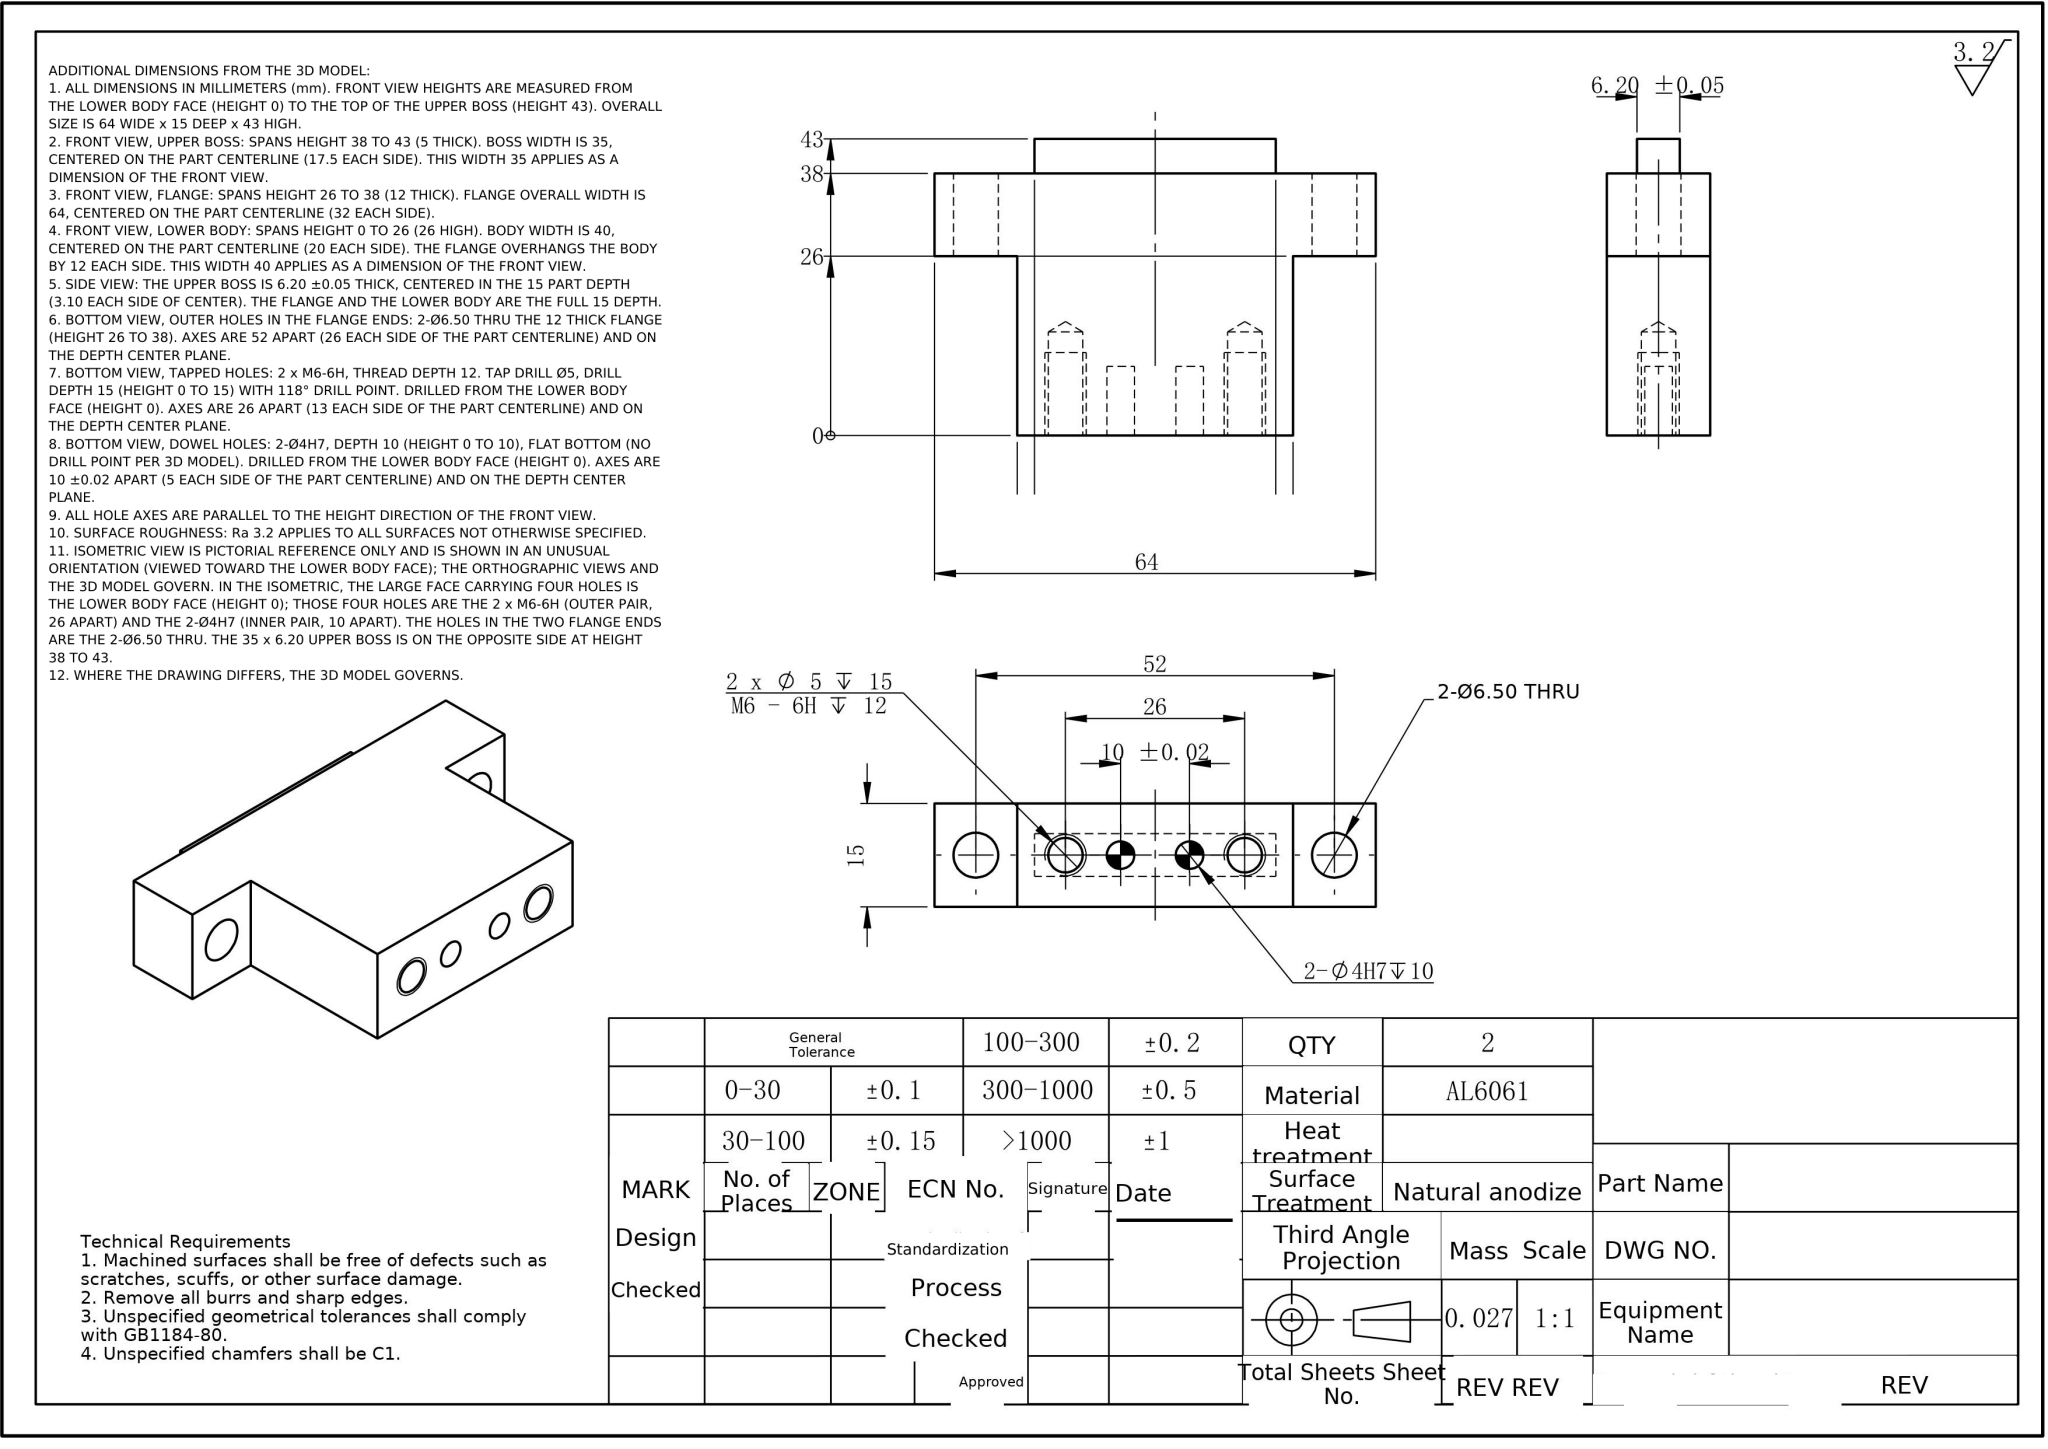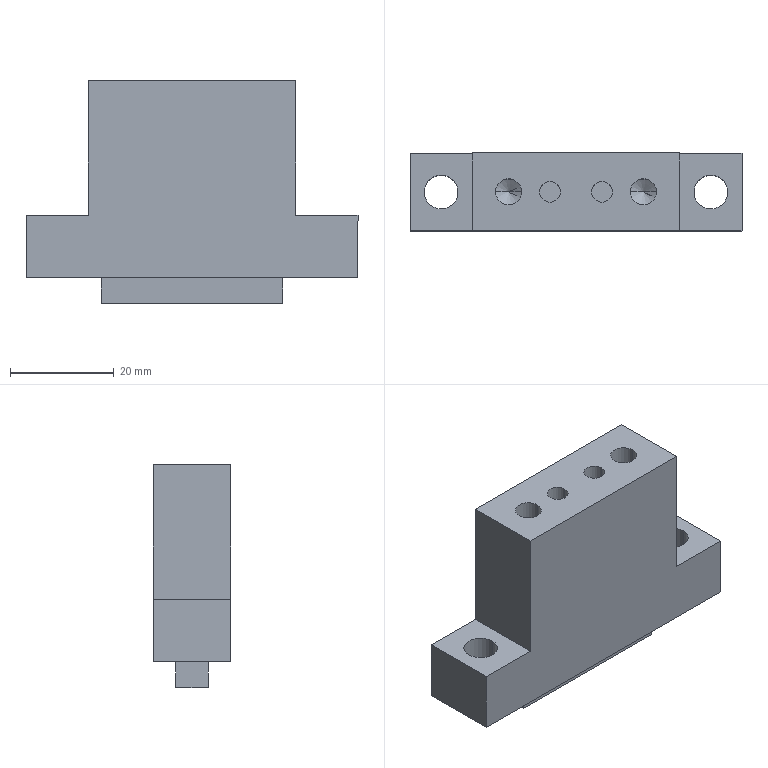Part | NX | mm | 1 solid | 33 faces | box 64 x 15 x 43 mm | volume 26549 mm3 | plane 17 | cylinder 12 | cone 4 | commonest cylinder face diameters 4 x4 5 x4 6.5 x4
STEP:
#1=CARTESIAN_POINT('',(-7.,-0.,-52.75));
#2=VERTEX_POINT('',#1);
#3=CARTESIAN_POINT('',(-3.,-0.,-52.75));
#4=VERTEX_POINT('',#3);
#5=CARTESIAN_POINT('',(-5.,-0.,-52.75));
#6=DIRECTION('',(0.,0.,1.));
#7=DIRECTION('',(-1.,0.,0.));
#8=AXIS2_PLACEMENT_3D('',#5,#6,#7);
#9=CIRCLE('',#8,2.);
#10=EDGE_CURVE('',#2,#4,#9,.T.);
#11=ORIENTED_EDGE('',*,*,#10,.F.);
#12=CARTESIAN_POINT('',(-7.,-0.,-42.75));
#13=VERTEX_POINT('',#12);
#14=CARTESIAN_POINT('',(-7.,-0.,-52.75));
#15=DIRECTION('',(0.,0.,1.));
#16=VECTOR('',#15,1000.);
#17=LINE('',#14,#16);
#18=EDGE_CURVE('',#2,#13,#17,.T.);
#19=ORIENTED_EDGE('',*,*,#18,.T.);
#20=CARTESIAN_POINT('',(-3.,-0.,-42.75));
#21=VERTEX_POINT('',#20);
#22=CARTESIAN_POINT('',(-5.,-0.,-42.75));
#23=DIRECTION('',(0.,0.,1.));
#24=DIRECTION('',(-1.,0.,0.));
#25=AXIS2_PLACEMENT_3D('',#22,#23,#24);
#26=CIRCLE('',#25,2.);
#27=EDGE_CURVE('',#13,#21,#26,.T.);
#28=ORIENTED_EDGE('',*,*,#27,.T.);
#29=CARTESIAN_POINT('',(-3.,-0.,-52.75));
#30=DIRECTION('',(0.,0.,1.));
#31=VECTOR('',#30,1000.);
#32=LINE('',#29,#31);
#33=EDGE_CURVE('',#4,#21,#32,.T.);
#34=ORIENTED_EDGE('',*,*,#33,.F.);
#35=EDGE_LOOP('',(#11,#19,#28,#34));
#36=FACE_OUTER_BOUND('',#35,.T.);
#37=CARTESIAN_POINT('',(-5.,-0.,-52.75));
#38=DIRECTION('',(0.,0.,1.));
#39=DIRECTION('',(1.,0.,0.));
#40=AXIS2_PLACEMENT_3D('',#37,#38,#39);
#41=CYLINDRICAL_SURFACE('',#40,2.);
#42=ADVANCED_FACE('',(#36),#41,.F.);
#43=CARTESIAN_POINT('',(3.,0.,-52.75));
#44=VERTEX_POINT('',#43);
#45=CARTESIAN_POINT('',(7.,0.,-52.75));
#46=VERTEX_POINT('',#45);
#47=CARTESIAN_POINT('',(5.,0.,-52.75));
#48=DIRECTION('',(0.,0.,1.));
#49=DIRECTION('',(1.,0.,0.));
#50=AXIS2_PLACEMENT_3D('',#47,#48,#49);
#51=CIRCLE('',#50,2.);
#52=EDGE_CURVE('',#44,#46,#51,.T.);
#53=ORIENTED_EDGE('',*,*,#52,.F.);
#54=CARTESIAN_POINT('',(3.,0.,-42.75));
#55=VERTEX_POINT('',#54);
#56=CARTESIAN_POINT('',(3.,0.,-52.75));
#57=DIRECTION('',(0.,0.,1.));
#58=VECTOR('',#57,1000.);
#59=LINE('',#56,#58);
#60=EDGE_CURVE('',#44,#55,#59,.T.);
#61=ORIENTED_EDGE('',*,*,#60,.T.);
#62=CARTESIAN_POINT('',(7.,0.,-42.75));
#63=VERTEX_POINT('',#62);
#64=CARTESIAN_POINT('',(5.,0.,-42.75));
#65=DIRECTION('',(0.,0.,1.));
#66=DIRECTION('',(1.,0.,0.));
#67=AXIS2_PLACEMENT_3D('',#64,#65,#66);
#68=CIRCLE('',#67,2.);
#69=EDGE_CURVE('',#55,#63,#68,.T.);
#70=ORIENTED_EDGE('',*,*,#69,.T.);
#71=CARTESIAN_POINT('',(7.,0.,-52.75));
#72=DIRECTION('',(0.,0.,1.));
#73=VECTOR('',#72,1000.);
#74=LINE('',#71,#73);
#75=EDGE_CURVE('',#46,#63,#74,.T.);
#76=ORIENTED_EDGE('',*,*,#75,.F.);
#77=EDGE_LOOP('',(#53,#61,#70,#76));
#78=FACE_OUTER_BOUND('',#77,.T.);
#79=CARTESIAN_POINT('',(5.,0.,-52.75));
#80=DIRECTION('',(0.,0.,1.));
#81=DIRECTION('',(1.,0.,0.));
#82=AXIS2_PLACEMENT_3D('',#79,#80,#81);
#83=CYLINDRICAL_SURFACE('',#82,2.);
#84=ADVANCED_FACE('',(#78),#83,.F.);
#85=CARTESIAN_POINT('',(10.5,0.,-57.75));
#86=VERTEX_POINT('',#85);
#87=CARTESIAN_POINT('',(15.5,0.,-57.75));
#88=VERTEX_POINT('',#87);
#89=CARTESIAN_POINT('',(13.,0.,-57.75));
#90=DIRECTION('',(0.,0.,1.));
#91=DIRECTION('',(1.,0.,0.));
#92=AXIS2_PLACEMENT_3D('',#89,#90,#91);
#93=CIRCLE('',#92,2.5);
#94=EDGE_CURVE('',#86,#88,#93,.T.);
#95=ORIENTED_EDGE('',*,*,#94,.F.);
#96=CARTESIAN_POINT('',(10.5,0.,-42.75));
#97=VERTEX_POINT('',#96);
#98=CARTESIAN_POINT('',(10.5,0.,-42.75));
#99=DIRECTION('',(0.,0.,1.));
#100=VECTOR('',#99,1000.);
#101=LINE('',#98,#100);
#102=EDGE_CURVE('',#86,#97,#101,.T.);
#103=ORIENTED_EDGE('',*,*,#102,.T.);
#104=CARTESIAN_POINT('',(15.5,0.,-42.75));
#105=VERTEX_POINT('',#104);
#106=CARTESIAN_POINT('',(13.,0.,-42.75));
#107=DIRECTION('',(0.,0.,1.));
#108=DIRECTION('',(1.,0.,0.));
#109=AXIS2_PLACEMENT_3D('',#106,#107,#108);
#110=CIRCLE('',#109,2.5);
#111=EDGE_CURVE('',#97,#105,#110,.T.);
#112=ORIENTED_EDGE('',*,*,#111,.T.);
#113=CARTESIAN_POINT('',(15.5,0.,-42.75));
#114=DIRECTION('',(0.,0.,1.));
#115=VECTOR('',#114,1000.);
#116=LINE('',#113,#115);
#117=EDGE_CURVE('',#88,#105,#116,.T.);
#118=ORIENTED_EDGE('',*,*,#117,.F.);
#119=EDGE_LOOP('',(#95,#103,#112,#118));
#120=FACE_OUTER_BOUND('',#119,.T.);
#121=CARTESIAN_POINT('',(13.,0.,-42.75));
#122=DIRECTION('',(0.,0.,1.));
#123=DIRECTION('',(1.,0.,0.));
#124=AXIS2_PLACEMENT_3D('',#121,#122,#123);
#125=CYLINDRICAL_SURFACE('',#124,2.5);
#126=ADVANCED_FACE('',(#120),#125,.F.);
#127=CARTESIAN_POINT('',(13.,0.,-59.252));
#128=VERTEX_POINT('',#127);
#129=CARTESIAN_POINT('',(15.5,0.,-57.75));
#130=DIRECTION('',(0.8572,0.,0.515));
#131=VECTOR('',#130,1000.);
#132=LINE('',#129,#131);
#133=EDGE_CURVE('',#128,#88,#132,.T.);
#134=ORIENTED_EDGE('',*,*,#133,.F.);
#135=CARTESIAN_POINT('',(10.5,0.,-57.75));
#136=DIRECTION('',(-0.8572,0.,0.515));
#137=VECTOR('',#136,1000.);
#138=LINE('',#135,#137);
#139=EDGE_CURVE('',#128,#86,#138,.T.);
#140=ORIENTED_EDGE('',*,*,#139,.T.);
#141=ORIENTED_EDGE('',*,*,#94,.T.);
#142=EDGE_LOOP('',(#134,#140,#141));
#143=FACE_OUTER_BOUND('',#142,.T.);
#144=CARTESIAN_POINT('',(13.,0.,-57.75));
#145=DIRECTION('',(0.,0.,1.));
#146=DIRECTION('',(1.,0.,0.));
#147=AXIS2_PLACEMENT_3D('',#144,#145,#146);
#148=CONICAL_SURFACE('',#147,2.5,1.03);
#149=ADVANCED_FACE('',(#143),#148,.F.);
#150=CARTESIAN_POINT('',(-15.5,0.,-57.75));
#151=VERTEX_POINT('',#150);
#152=CARTESIAN_POINT('',(-10.5,0.,-57.75));
#153=VERTEX_POINT('',#152);
#154=CARTESIAN_POINT('',(-13.,0.,-57.75));
#155=DIRECTION('',(0.,0.,1.));
#156=DIRECTION('',(1.,0.,0.));
#157=AXIS2_PLACEMENT_3D('',#154,#155,#156);
#158=CIRCLE('',#157,2.5);
#159=EDGE_CURVE('',#151,#153,#158,.T.);
#160=ORIENTED_EDGE('',*,*,#159,.F.);
#161=CARTESIAN_POINT('',(-15.5,0.,-42.75));
#162=VERTEX_POINT('',#161);
#163=CARTESIAN_POINT('',(-15.5,0.,-42.75));
#164=DIRECTION('',(0.,0.,1.));
#165=VECTOR('',#164,1000.);
#166=LINE('',#163,#165);
#167=EDGE_CURVE('',#151,#162,#166,.T.);
#168=ORIENTED_EDGE('',*,*,#167,.T.);
#169=CARTESIAN_POINT('',(-10.5,0.,-42.75));
#170=VERTEX_POINT('',#169);
#171=CARTESIAN_POINT('',(-13.,0.,-42.75));
#172=DIRECTION('',(0.,0.,1.));
#173=DIRECTION('',(1.,0.,0.));
#174=AXIS2_PLACEMENT_3D('',#171,#172,#173);
#175=CIRCLE('',#174,2.5);
#176=EDGE_CURVE('',#162,#170,#175,.T.);
#177=ORIENTED_EDGE('',*,*,#176,.T.);
#178=CARTESIAN_POINT('',(-10.5,0.,-42.75));
#179=DIRECTION('',(0.,0.,1.));
#180=VECTOR('',#179,1000.);
#181=LINE('',#178,#180);
#182=EDGE_CURVE('',#153,#170,#181,.T.);
#183=ORIENTED_EDGE('',*,*,#182,.F.);
#184=EDGE_LOOP('',(#160,#168,#177,#183));
#185=FACE_OUTER_BOUND('',#184,.T.);
#186=CARTESIAN_POINT('',(-13.,0.,-42.75));
#187=DIRECTION('',(0.,0.,1.));
#188=DIRECTION('',(1.,0.,0.));
#189=AXIS2_PLACEMENT_3D('',#186,#187,#188);
#190=CYLINDRICAL_SURFACE('',#189,2.5);
#191=ADVANCED_FACE('',(#185),#190,.F.);
#192=CARTESIAN_POINT('',(-13.,0.,-59.252));
#193=VERTEX_POINT('',#192);
#194=CARTESIAN_POINT('',(-10.5,0.,-57.75));
#195=DIRECTION('',(0.8572,0.,0.515));
#196=VECTOR('',#195,1000.);
#197=LINE('',#194,#196);
#198=EDGE_CURVE('',#193,#153,#197,.T.);
#199=ORIENTED_EDGE('',*,*,#198,.F.);
#200=CARTESIAN_POINT('',(-15.5,0.,-57.75));
#201=DIRECTION('',(-0.8572,0.,0.515));
#202=VECTOR('',#201,1000.);
#203=LINE('',#200,#202);
#204=EDGE_CURVE('',#193,#151,#203,.T.);
#205=ORIENTED_EDGE('',*,*,#204,.T.);
#206=ORIENTED_EDGE('',*,*,#159,.T.);
#207=EDGE_LOOP('',(#199,#205,#206));
#208=FACE_OUTER_BOUND('',#207,.T.);
#209=CARTESIAN_POINT('',(-13.,0.,-57.75));
#210=DIRECTION('',(0.,0.,1.));
#211=DIRECTION('',(1.,0.,0.));
#212=AXIS2_PLACEMENT_3D('',#209,#210,#211);
#213=CONICAL_SURFACE('',#212,2.5,1.03);
#214=ADVANCED_FACE('',(#208),#213,.F.);
#215=CARTESIAN_POINT('',(29.25,-0.,-68.75));
#216=VERTEX_POINT('',#215);
#217=CARTESIAN_POINT('',(22.75,-0.,-68.75));
#218=VERTEX_POINT('',#217);
#219=CARTESIAN_POINT('',(26.,-0.,-68.75));
#220=DIRECTION('',(0.,0.,-1.));
#221=DIRECTION('',(-1.,0.,0.));
#222=AXIS2_PLACEMENT_3D('',#219,#220,#221);
#223=CIRCLE('',#222,3.25);
#224=EDGE_CURVE('',#216,#218,#223,.T.);
#225=ORIENTED_EDGE('',*,*,#224,.F.);
#226=CARTESIAN_POINT('',(29.25,-0.,-80.75));
#227=VERTEX_POINT('',#226);
#228=CARTESIAN_POINT('',(29.25,-0.,89.942));
#229=DIRECTION('',(0.,0.,-1.));
#230=VECTOR('',#229,1000.);
#231=LINE('',#228,#230);
#232=EDGE_CURVE('',#216,#227,#231,.T.);
#233=ORIENTED_EDGE('',*,*,#232,.T.);
#234=CARTESIAN_POINT('',(22.75,-0.,-80.75));
#235=VERTEX_POINT('',#234);
#236=CARTESIAN_POINT('',(26.,-0.,-80.75));
#237=DIRECTION('',(0.,0.,-1.));
#238=DIRECTION('',(1.,0.,0.));
#239=AXIS2_PLACEMENT_3D('',#236,#237,#238);
#240=CIRCLE('',#239,3.25);
#241=EDGE_CURVE('',#227,#235,#240,.T.);
#242=ORIENTED_EDGE('',*,*,#241,.T.);
#243=CARTESIAN_POINT('',(22.75,-0.,89.942));
#244=DIRECTION('',(0.,0.,-1.));
#245=VECTOR('',#244,1000.);
#246=LINE('',#243,#245);
#247=EDGE_CURVE('',#218,#235,#246,.T.);
#248=ORIENTED_EDGE('',*,*,#247,.F.);
#249=EDGE_LOOP('',(#225,#233,#242,#248));
#250=FACE_OUTER_BOUND('',#249,.T.);
#251=CARTESIAN_POINT('',(26.,-0.,89.942));
#252=DIRECTION('',(0.,0.,-1.));
#253=DIRECTION('',(-1.,0.,0.));
#254=AXIS2_PLACEMENT_3D('',#251,#252,#253);
#255=CYLINDRICAL_SURFACE('',#254,3.25);
#256=ADVANCED_FACE('',(#250),#255,.F.);
#257=CARTESIAN_POINT('',(-22.75,0.,-68.75));
#258=VERTEX_POINT('',#257);
#259=CARTESIAN_POINT('',(-29.25,0.,-68.75));
#260=VERTEX_POINT('',#259);
#261=CARTESIAN_POINT('',(-26.,0.,-68.75));
#262=DIRECTION('',(0.,0.,-1.));
#263=DIRECTION('',(-1.,0.,0.));
#264=AXIS2_PLACEMENT_3D('',#261,#262,#263);
#265=CIRCLE('',#264,3.25);
#266=EDGE_CURVE('',#258,#260,#265,.T.);
#267=ORIENTED_EDGE('',*,*,#266,.F.);
#268=CARTESIAN_POINT('',(-22.75,0.,-80.75));
#269=VERTEX_POINT('',#268);
#270=CARTESIAN_POINT('',(-22.75,0.,89.942));
#271=DIRECTION('',(0.,0.,-1.));
#272=VECTOR('',#271,1000.);
#273=LINE('',#270,#272);
#274=EDGE_CURVE('',#258,#269,#273,.T.);
#275=ORIENTED_EDGE('',*,*,#274,.T.);
#276=CARTESIAN_POINT('',(-29.25,0.,-80.75));
#277=VERTEX_POINT('',#276);
#278=CARTESIAN_POINT('',(-26.,0.,-80.75));
#279=DIRECTION('',(0.,0.,-1.));
#280=DIRECTION('',(-1.,0.,0.));
#281=AXIS2_PLACEMENT_3D('',#278,#279,#280);
#282=CIRCLE('',#281,3.25);
#283=EDGE_CURVE('',#269,#277,#282,.T.);
#284=ORIENTED_EDGE('',*,*,#283,.T.);
#285=CARTESIAN_POINT('',(-29.25,0.,89.942));
#286=DIRECTION('',(0.,0.,-1.));
#287=VECTOR('',#286,1000.);
#288=LINE('',#285,#287);
#289=EDGE_CURVE('',#260,#277,#288,.T.);
#290=ORIENTED_EDGE('',*,*,#289,.F.);
#291=EDGE_LOOP('',(#267,#275,#284,#290));
#292=FACE_OUTER_BOUND('',#291,.T.);
#293=CARTESIAN_POINT('',(-26.,0.,89.942));
#294=DIRECTION('',(0.,0.,-1.));
#295=DIRECTION('',(-1.,0.,0.));
#296=AXIS2_PLACEMENT_3D('',#293,#294,#295);
#297=CYLINDRICAL_SURFACE('',#296,3.25);
#298=ADVANCED_FACE('',(#292),#297,.F.);
#299=CARTESIAN_POINT('',(26.,-0.,-80.75));
#300=DIRECTION('',(0.,0.,-1.));
#301=DIRECTION('',(1.,0.,0.));
#302=AXIS2_PLACEMENT_3D('',#299,#300,#301);
#303=CIRCLE('',#302,3.25);
#304=EDGE_CURVE('',#235,#227,#303,.T.);
#305=ORIENTED_EDGE('',*,*,#304,.F.);
#306=ORIENTED_EDGE('',*,*,#241,.F.);
#307=EDGE_LOOP('',(#305,#306));
#308=FACE_BOUND('',#307,.T.);
#309=CARTESIAN_POINT('',(-26.,0.,-80.75));
#310=DIRECTION('',(0.,0.,-1.));
#311=DIRECTION('',(-1.,0.,0.));
#312=AXIS2_PLACEMENT_3D('',#309,#310,#311);
#313=CIRCLE('',#312,3.25);
#314=EDGE_CURVE('',#277,#269,#313,.T.);
#315=ORIENTED_EDGE('',*,*,#314,.F.);
#316=ORIENTED_EDGE('',*,*,#283,.F.);
#317=EDGE_LOOP('',(#315,#316));
#318=FACE_BOUND('',#317,.T.);
#319=CARTESIAN_POINT('',(32.,-7.5,-80.75));
#320=VERTEX_POINT('',#319);
#321=CARTESIAN_POINT('',(-32.,-7.5,-80.75));
#322=VERTEX_POINT('',#321);
#323=CARTESIAN_POINT('',(-32.,-7.5,-80.75));
#324=DIRECTION('',(-1.,0.,0.));
#325=VECTOR('',#324,1000.);
#326=LINE('',#323,#325);
#327=EDGE_CURVE('',#320,#322,#326,.T.);
#328=ORIENTED_EDGE('',*,*,#327,.T.);
#329=CARTESIAN_POINT('',(-32.,7.5,-80.75));
#330=VERTEX_POINT('',#329);
#331=CARTESIAN_POINT('',(-32.,7.5,-80.75));
#332=DIRECTION('',(0.,-1.,0.));
#333=VECTOR('',#332,1000.);
#334=LINE('',#331,#333);
#335=EDGE_CURVE('',#330,#322,#334,.T.);
#336=ORIENTED_EDGE('',*,*,#335,.F.);
#337=CARTESIAN_POINT('',(32.,7.5,-80.75));
#338=VERTEX_POINT('',#337);
#339=CARTESIAN_POINT('',(-32.,7.5,-80.75));
#340=DIRECTION('',(-1.,0.,0.));
#341=VECTOR('',#340,1000.);
#342=LINE('',#339,#341);
#343=EDGE_CURVE('',#338,#330,#342,.T.);
#344=ORIENTED_EDGE('',*,*,#343,.F.);
#345=CARTESIAN_POINT('',(32.,7.5,-80.75));
#346=DIRECTION('',(0.,-1.,0.));
#347=VECTOR('',#346,1000.);
#348=LINE('',#345,#347);
#349=EDGE_CURVE('',#338,#320,#348,.T.);
#350=ORIENTED_EDGE('',*,*,#349,.T.);
#351=EDGE_LOOP('',(#328,#336,#344,#350));
#352=FACE_OUTER_BOUND('',#351,.T.);
#353=CARTESIAN_POINT('',(-17.5,-3.1,-80.75));
#354=VERTEX_POINT('',#353);
#355=CARTESIAN_POINT('',(-17.5,3.1,-80.75));
#356=VERTEX_POINT('',#355);
#357=CARTESIAN_POINT('',(-17.5,-3.1,-80.75));
#358=DIRECTION('',(0.,1.,0.));
#359=VECTOR('',#358,1000.);
#360=LINE('',#357,#359);
#361=EDGE_CURVE('',#354,#356,#360,.T.);
#362=ORIENTED_EDGE('',*,*,#361,.F.);
#363=CARTESIAN_POINT('',(17.5,-3.1,-80.75));
#364=VERTEX_POINT('',#363);
#365=CARTESIAN_POINT('',(17.5,-3.1,-80.75));
#366=DIRECTION('',(-1.,0.,0.));
#367=VECTOR('',#366,1000.);
#368=LINE('',#365,#367);
#369=EDGE_CURVE('',#364,#354,#368,.T.);
#370=ORIENTED_EDGE('',*,*,#369,.F.);
#371=CARTESIAN_POINT('',(17.5,3.1,-80.75));
#372=VERTEX_POINT('',#371);
#373=CARTESIAN_POINT('',(17.5,-3.1,-80.75));
#374=DIRECTION('',(0.,-1.,0.));
#375=VECTOR('',#374,1000.);
#376=LINE('',#373,#375);
#377=EDGE_CURVE('',#372,#364,#376,.T.);
#378=ORIENTED_EDGE('',*,*,#377,.F.);
#379=CARTESIAN_POINT('',(17.5,3.1,-80.75));
#380=DIRECTION('',(1.,0.,0.));
#381=VECTOR('',#380,1000.);
#382=LINE('',#379,#381);
#383=EDGE_CURVE('',#356,#372,#382,.T.);
#384=ORIENTED_EDGE('',*,*,#383,.F.);
#385=EDGE_LOOP('',(#362,#370,#378,#384));
#386=FACE_BOUND('',#385,.T.);
#387=CARTESIAN_POINT('',(-32.,7.5,-80.75));
#388=DIRECTION('',(0.,0.,1.));
#389=DIRECTION('',(1.,0.,0.));
#390=AXIS2_PLACEMENT_3D('',#387,#388,#389);
#391=PLANE('',#390);
#392=ADVANCED_FACE('',(#308,#318,#352,#386),#391,.F.);
#393=CARTESIAN_POINT('',(32.,7.5,-68.75));
#394=VERTEX_POINT('',#393);
#395=CARTESIAN_POINT('',(32.,7.5,80.75));
#396=DIRECTION('',(0.,0.,-1.));
#397=VECTOR('',#396,1000.);
#398=LINE('',#395,#397);
#399=EDGE_CURVE('',#394,#338,#398,.T.);
#400=ORIENTED_EDGE('',*,*,#399,.F.);
#401=CARTESIAN_POINT('',(32.,-7.5,-68.75));
#402=VERTEX_POINT('',#401);
#403=CARTESIAN_POINT('',(32.,12.5,-68.75));
#404=DIRECTION('',(0.,-1.,0.));
#405=VECTOR('',#404,1000.);
#406=LINE('',#403,#405);
#407=EDGE_CURVE('',#394,#402,#406,.T.);
#408=ORIENTED_EDGE('',*,*,#407,.T.);
#409=CARTESIAN_POINT('',(32.,-7.5,80.75));
#410=DIRECTION('',(0.,0.,-1.));
#411=VECTOR('',#410,1000.);
#412=LINE('',#409,#411);
#413=EDGE_CURVE('',#402,#320,#412,.T.);
#414=ORIENTED_EDGE('',*,*,#413,.T.);
#415=ORIENTED_EDGE('',*,*,#349,.F.);
#416=EDGE_LOOP('',(#400,#408,#414,#415));
#417=FACE_OUTER_BOUND('',#416,.T.);
#418=CARTESIAN_POINT('',(32.,7.5,80.75));
#419=DIRECTION('',(-1.,0.,0.));
#420=DIRECTION('',(0.,0.,1.));
#421=AXIS2_PLACEMENT_3D('',#418,#419,#420);
#422=PLANE('',#421);
#423=ADVANCED_FACE('',(#417),#422,.F.);
#424=CARTESIAN_POINT('',(-32.,-7.5,-68.75));
#425=VERTEX_POINT('',#424);
#426=CARTESIAN_POINT('',(-32.,-7.5,80.75));
#427=DIRECTION('',(0.,0.,1.));
#428=VECTOR('',#427,1000.);
#429=LINE('',#426,#428);
#430=EDGE_CURVE('',#322,#425,#429,.T.);
#431=ORIENTED_EDGE('',*,*,#430,.T.);
#432=CARTESIAN_POINT('',(-32.,7.5,-68.75));
#433=VERTEX_POINT('',#432);
#434=CARTESIAN_POINT('',(-32.,12.5,-68.75));
#435=DIRECTION('',(0.,-1.,0.));
#436=VECTOR('',#435,1000.);
#437=LINE('',#434,#436);
#438=EDGE_CURVE('',#433,#425,#437,.T.);
#439=ORIENTED_EDGE('',*,*,#438,.F.);
#440=CARTESIAN_POINT('',(-32.,7.5,80.75));
#441=DIRECTION('',(0.,0.,1.));
#442=VECTOR('',#441,1000.);
#443=LINE('',#440,#442);
#444=EDGE_CURVE('',#330,#433,#443,.T.);
#445=ORIENTED_EDGE('',*,*,#444,.F.);
#446=ORIENTED_EDGE('',*,*,#335,.T.);
#447=EDGE_LOOP('',(#431,#439,#445,#446));
#448=FACE_OUTER_BOUND('',#447,.T.);
#449=CARTESIAN_POINT('',(-32.,7.5,80.75));
#450=DIRECTION('',(1.,0.,0.));
#451=DIRECTION('',(0.,0.,-1.));
#452=AXIS2_PLACEMENT_3D('',#449,#450,#451);
#453=PLANE('',#452);
#454=ADVANCED_FACE('',(#448),#453,.F.);
#455=CARTESIAN_POINT('',(-20.,7.5,-68.75));
#456=VERTEX_POINT('',#455);
#457=CARTESIAN_POINT('',(-20.,7.5,-42.75));
#458=VERTEX_POINT('',#457);
#459=CARTESIAN_POINT('',(-20.,7.5,-0.));
#460=DIRECTION('',(-0.,0.,1.));
#461=VECTOR('',#460,1000.);
#462=LINE('',#459,#461);
#463=EDGE_CURVE('',#456,#458,#462,.T.);
#464=ORIENTED_EDGE('',*,*,#463,.T.);
#465=CARTESIAN_POINT('',(20.,7.5,-42.75));
#466=VERTEX_POINT('',#465);
#467=CARTESIAN_POINT('',(0.,7.5,-42.75));
#468=DIRECTION('',(1.,0.,0.));
#469=VECTOR('',#468,1000.);
#470=LINE('',#467,#469);
#471=EDGE_CURVE('',#458,#466,#470,.T.);
#472=ORIENTED_EDGE('',*,*,#471,.T.);
#473=CARTESIAN_POINT('',(20.,7.5,-68.75));
#474=VERTEX_POINT('',#473);
#475=CARTESIAN_POINT('',(20.,7.5,0.));
#476=DIRECTION('',(0.,0.,-1.));
#477=VECTOR('',#476,1000.);
#478=LINE('',#475,#477);
#479=EDGE_CURVE('',#466,#474,#478,.T.);
#480=ORIENTED_EDGE('',*,*,#479,.T.);
#481=CARTESIAN_POINT('',(0.,7.5,-68.75));
#482=DIRECTION('',(1.,0.,0.));
#483=VECTOR('',#482,1000.);
#484=LINE('',#481,#483);
#485=EDGE_CURVE('',#474,#394,#484,.T.);
#486=ORIENTED_EDGE('',*,*,#485,.T.);
#487=ORIENTED_EDGE('',*,*,#399,.T.);
#488=ORIENTED_EDGE('',*,*,#343,.T.);
#489=ORIENTED_EDGE('',*,*,#444,.T.);
#490=CARTESIAN_POINT('',(0.,7.5,-68.75));
#491=DIRECTION('',(1.,0.,0.));
#492=VECTOR('',#491,1000.);
#493=LINE('',#490,#492);
#494=EDGE_CURVE('',#433,#456,#493,.T.);
#495=ORIENTED_EDGE('',*,*,#494,.T.);
#496=EDGE_LOOP('',(#464,#472,#480,#486,#487,#488,#489,#495));
#497=FACE_OUTER_BOUND('',#496,.T.);
#498=CARTESIAN_POINT('',(0.,7.5,0.));
#499=DIRECTION('',(0.,-1.,0.));
#500=DIRECTION('',(0.,0.,-1.));
#501=AXIS2_PLACEMENT_3D('',#498,#499,#500);
#502=PLANE('',#501);
#503=ADVANCED_FACE('',(#497),#502,.F.);
#504=CARTESIAN_POINT('',(-20.,-7.5,-42.75));
#505=VERTEX_POINT('',#504);
#506=CARTESIAN_POINT('',(20.,-7.5,-42.75));
#507=VERTEX_POINT('',#506);
#508=CARTESIAN_POINT('',(-32.,-7.5,-42.75));
#509=DIRECTION('',(1.,0.,0.));
#510=VECTOR('',#509,1000.);
#511=LINE('',#508,#510);
#512=EDGE_CURVE('',#505,#507,#511,.T.);
#513=ORIENTED_EDGE('',*,*,#512,.F.);
#514=CARTESIAN_POINT('',(-20.,-7.5,-68.75));
#515=VERTEX_POINT('',#514);
#516=CARTESIAN_POINT('',(-20.,-7.5,-68.75));
#517=DIRECTION('',(-0.,0.,1.));
#518=VECTOR('',#517,1000.);
#519=LINE('',#516,#518);
#520=EDGE_CURVE('',#515,#505,#519,.T.);
#521=ORIENTED_EDGE('',*,*,#520,.F.);
#522=CARTESIAN_POINT('',(-32.,-7.5,-68.75));
#523=DIRECTION('',(1.,0.,0.));
#524=VECTOR('',#523,1000.);
#525=LINE('',#522,#524);
#526=EDGE_CURVE('',#425,#515,#525,.T.);
#527=ORIENTED_EDGE('',*,*,#526,.F.);
#528=ORIENTED_EDGE('',*,*,#430,.F.);
#529=ORIENTED_EDGE('',*,*,#327,.F.);
#530=ORIENTED_EDGE('',*,*,#413,.F.);
#531=CARTESIAN_POINT('',(20.,-7.5,-68.75));
#532=VERTEX_POINT('',#531);
#533=CARTESIAN_POINT('',(32.,-7.5,-68.75));
#534=DIRECTION('',(1.,0.,0.));
#535=VECTOR('',#534,1000.);
#536=LINE('',#533,#535);
#537=EDGE_CURVE('',#532,#402,#536,.T.);
#538=ORIENTED_EDGE('',*,*,#537,.F.);
#539=CARTESIAN_POINT('',(20.,-7.5,-68.75));
#540=DIRECTION('',(0.,0.,-1.));
#541=VECTOR('',#540,1000.);
#542=LINE('',#539,#541);
#543=EDGE_CURVE('',#507,#532,#542,.T.);
#544=ORIENTED_EDGE('',*,*,#543,.F.);
#545=EDGE_LOOP('',(#513,#521,#527,#528,#529,#530,#538,#544));
#546=FACE_OUTER_BOUND('',#545,.T.);
#547=CARTESIAN_POINT('',(0.,-7.5,0.));
#548=DIRECTION('',(0.,-1.,0.));
#549=DIRECTION('',(0.,0.,-1.));
#550=AXIS2_PLACEMENT_3D('',#547,#548,#549);
#551=PLANE('',#550);
#552=ADVANCED_FACE('',(#546),#551,.T.);
#553=ORIENTED_EDGE('',*,*,#520,.T.);
#554=CARTESIAN_POINT('',(-20.,12.5,-42.75));
#555=DIRECTION('',(0.,1.,0.));
#556=VECTOR('',#555,1000.);
#557=LINE('',#554,#556);
#558=EDGE_CURVE('',#505,#458,#557,.T.);
#559=ORIENTED_EDGE('',*,*,#558,.T.);
#560=ORIENTED_EDGE('',*,*,#463,.F.);
#561=CARTESIAN_POINT('',(-20.,12.5,-68.75));
#562=DIRECTION('',(0.,-1.,0.));
#563=VECTOR('',#562,1000.);
#564=LINE('',#561,#563);
#565=EDGE_CURVE('',#456,#515,#564,.T.);
#566=ORIENTED_EDGE('',*,*,#565,.T.);
#567=EDGE_LOOP('',(#553,#559,#560,#566));
#568=FACE_OUTER_BOUND('',#567,.T.);
#569=CARTESIAN_POINT('',(-20.,12.5,-68.75));
#570=DIRECTION('',(1.,0.,0.));
#571=DIRECTION('',(0.,0.,-1.));
#572=AXIS2_PLACEMENT_3D('',#569,#570,#571);
#573=PLANE('',#572);
#574=ADVANCED_FACE('',(#568),#573,.F.);
#575=CARTESIAN_POINT('',(-26.,0.,-68.75));
#576=DIRECTION('',(0.,0.,-1.));
#577=DIRECTION('',(-1.,0.,0.));
#578=AXIS2_PLACEMENT_3D('',#575,#576,#577);
#579=CIRCLE('',#578,3.25);
#580=EDGE_CURVE('',#260,#258,#579,.T.);
#581=ORIENTED_EDGE('',*,*,#580,.T.);
#582=ORIENTED_EDGE('',*,*,#266,.T.);
#583=EDGE_LOOP('',(#581,#582));
#584=FACE_BOUND('',#583,.T.);
#585=ORIENTED_EDGE('',*,*,#438,.T.);
#586=ORIENTED_EDGE('',*,*,#526,.T.);
#587=ORIENTED_EDGE('',*,*,#565,.F.);
#588=ORIENTED_EDGE('',*,*,#494,.F.);
#589=EDGE_LOOP('',(#585,#586,#587,#588));
#590=FACE_OUTER_BOUND('',#589,.T.);
#591=CARTESIAN_POINT('',(-32.,12.5,-68.75));
#592=DIRECTION('',(0.,0.,-1.));
#593=DIRECTION('',(-1.,0.,0.));
#594=AXIS2_PLACEMENT_3D('',#591,#592,#593);
#595=PLANE('',#594);
#596=ADVANCED_FACE('',(#584,#590),#595,.F.);
#597=CARTESIAN_POINT('',(26.,-0.,-68.75));
#598=DIRECTION('',(0.,0.,-1.));
#599=DIRECTION('',(-1.,0.,0.));
#600=AXIS2_PLACEMENT_3D('',#597,#598,#599);
#601=CIRCLE('',#600,3.25);
#602=EDGE_CURVE('',#218,#216,#601,.T.);
#603=ORIENTED_EDGE('',*,*,#602,.T.);
#604=ORIENTED_EDGE('',*,*,#224,.T.);
#605=EDGE_LOOP('',(#603,#604));
#606=FACE_BOUND('',#605,.T.);
#607=CARTESIAN_POINT('',(20.,12.5,-68.75));
#608=DIRECTION('',(0.,-1.,0.));
#609=VECTOR('',#608,1000.);
#610=LINE('',#607,#609);
#611=EDGE_CURVE('',#474,#532,#610,.T.);
#612=ORIENTED_EDGE('',*,*,#611,.T.);
#613=ORIENTED_EDGE('',*,*,#537,.T.);
#614=ORIENTED_EDGE('',*,*,#407,.F.);
#615=ORIENTED_EDGE('',*,*,#485,.F.);
#616=EDGE_LOOP('',(#612,#613,#614,#615));
#617=FACE_OUTER_BOUND('',#616,.T.);
#618=CARTESIAN_POINT('',(32.,12.5,-68.75));
#619=DIRECTION('',(0.,0.,-1.));
#620=DIRECTION('',(-1.,0.,-0.));
#621=AXIS2_PLACEMENT_3D('',#618,#619,#620);
#622=PLANE('',#621);
#623=ADVANCED_FACE('',(#606,#617),#622,.F.);
#624=ORIENTED_EDGE('',*,*,#479,.F.);
#625=CARTESIAN_POINT('',(20.,12.5,-42.75));
#626=DIRECTION('',(0.,-1.,0.));
#627=VECTOR('',#626,1000.);
#628=LINE('',#625,#627);
#629=EDGE_CURVE('',#466,#507,#628,.T.);
#630=ORIENTED_EDGE('',*,*,#629,.T.);
#631=ORIENTED_EDGE('',*,*,#543,.T.);
#632=ORIENTED_EDGE('',*,*,#611,.F.);
#633=EDGE_LOOP('',(#624,#630,#631,#632));
#634=FACE_OUTER_BOUND('',#633,.T.);
#635=CARTESIAN_POINT('',(20.,12.5,-68.75));
#636=DIRECTION('',(-1.,0.,-0.));
#637=DIRECTION('',(-0.,0.,1.));
#638=AXIS2_PLACEMENT_3D('',#635,#636,#637);
#639=PLANE('',#638);
#640=ADVANCED_FACE('',(#634),#639,.F.);
#641=ORIENTED_EDGE('',*,*,#361,.T.);
#642=CARTESIAN_POINT('',(-17.5,3.1,-85.75));
#643=VERTEX_POINT('',#642);
#644=CARTESIAN_POINT('',(-17.5,3.1,-85.75));
#645=DIRECTION('',(0.,0.,1.));
#646=VECTOR('',#645,1000.);
#647=LINE('',#644,#646);
#648=EDGE_CURVE('',#643,#356,#647,.T.);
#649=ORIENTED_EDGE('',*,*,#648,.F.);
#650=CARTESIAN_POINT('',(-17.5,-3.1,-85.75));
#651=VERTEX_POINT('',#650);
#652=CARTESIAN_POINT('',(-17.5,-3.1,-85.75));
#653=DIRECTION('',(0.,1.,0.));
#654=VECTOR('',#653,1000.);
#655=LINE('',#652,#654);
#656=EDGE_CURVE('',#651,#643,#655,.T.);
#657=ORIENTED_EDGE('',*,*,#656,.F.);
#658=CARTESIAN_POINT('',(-17.5,-3.1,-85.75));
#659=DIRECTION('',(0.,0.,1.));
#660=VECTOR('',#659,1000.);
#661=LINE('',#658,#660);
#662=EDGE_CURVE('',#651,#354,#661,.T.);
#663=ORIENTED_EDGE('',*,*,#662,.T.);
#664=EDGE_LOOP('',(#641,#649,#657,#663));
#665=FACE_OUTER_BOUND('',#664,.T.);
#666=CARTESIAN_POINT('',(-17.5,-3.1,-85.75));
#667=DIRECTION('',(1.,0.,0.));
#668=DIRECTION('',(0.,0.,-1.));
#669=AXIS2_PLACEMENT_3D('',#666,#667,#668);
#670=PLANE('',#669);
#671=ADVANCED_FACE('',(#665),#670,.F.);
#672=ORIENTED_EDGE('',*,*,#383,.T.);
#673=CARTESIAN_POINT('',(17.5,3.1,-85.75));
#674=VERTEX_POINT('',#673);
#675=CARTESIAN_POINT('',(17.5,3.1,-85.75));
#676=DIRECTION('',(0.,0.,1.));
#677=VECTOR('',#676,1000.);
#678=LINE('',#675,#677);
#679=EDGE_CURVE('',#674,#372,#678,.T.);
#680=ORIENTED_EDGE('',*,*,#679,.F.);
#681=CARTESIAN_POINT('',(17.5,3.1,-85.75));
#682=DIRECTION('',(1.,0.,0.));
#683=VECTOR('',#682,1000.);
#684=LINE('',#681,#683);
#685=EDGE_CURVE('',#643,#674,#684,.T.);
#686=ORIENTED_EDGE('',*,*,#685,.F.);
#687=ORIENTED_EDGE('',*,*,#648,.T.);
#688=EDGE_LOOP('',(#672,#680,#686,#687));
#689=FACE_OUTER_BOUND('',#688,.T.);
#690=CARTESIAN_POINT('',(17.5,3.1,-85.75));
#691=DIRECTION('',(0.,-1.,0.));
#692=DIRECTION('',(0.,0.,-1.));
#693=AXIS2_PLACEMENT_3D('',#690,#691,#692);
#694=PLANE('',#693);
#695=ADVANCED_FACE('',(#689),#694,.F.);
#696=ORIENTED_EDGE('',*,*,#377,.T.);
#697=CARTESIAN_POINT('',(17.5,-3.1,-85.75));
#698=VERTEX_POINT('',#697);
#699=CARTESIAN_POINT('',(17.5,-3.1,-85.75));
#700=DIRECTION('',(0.,0.,1.));
#701=VECTOR('',#700,1000.);
#702=LINE('',#699,#701);
#703=EDGE_CURVE('',#698,#364,#702,.T.);
#704=ORIENTED_EDGE('',*,*,#703,.F.);
#705=CARTESIAN_POINT('',(17.5,-3.1,-85.75));
#706=DIRECTION('',(0.,-1.,0.));
#707=VECTOR('',#706,1000.);
#708=LINE('',#705,#707);
#709=EDGE_CURVE('',#674,#698,#708,.T.);
#710=ORIENTED_EDGE('',*,*,#709,.F.);
#711=ORIENTED_EDGE('',*,*,#679,.T.);
#712=EDGE_LOOP('',(#696,#704,#710,#711));
#713=FACE_OUTER_BOUND('',#712,.T.);
#714=CARTESIAN_POINT('',(17.5,-3.1,-85.75));
#715=DIRECTION('',(-1.,0.,0.));
#716=DIRECTION('',(0.,0.,1.));
#717=AXIS2_PLACEMENT_3D('',#714,#715,#716);
#718=PLANE('',#717);
#719=ADVANCED_FACE('',(#713),#718,.F.);
#720=ORIENTED_EDGE('',*,*,#369,.T.);
#721=ORIENTED_EDGE('',*,*,#662,.F.);
#722=CARTESIAN_POINT('',(17.5,-3.1,-85.75));
#723=DIRECTION('',(-1.,0.,0.));
#724=VECTOR('',#723,1000.);
#725=LINE('',#722,#724);
#726=EDGE_CURVE('',#698,#651,#725,.T.);
#727=ORIENTED_EDGE('',*,*,#726,.F.);
#728=ORIENTED_EDGE('',*,*,#703,.T.);
#729=EDGE_LOOP('',(#720,#721,#727,#728));
#730=FACE_OUTER_BOUND('',#729,.T.);
#731=CARTESIAN_POINT('',(17.5,-3.1,-85.75));
#732=DIRECTION('',(0.,1.,0.));
#733=DIRECTION('',(0.,0.,1.));
#734=AXIS2_PLACEMENT_3D('',#731,#732,#733);
#735=PLANE('',#734);
#736=ADVANCED_FACE('',(#730),#735,.F.);
#737=ORIENTED_EDGE('',*,*,#656,.T.);
#738=ORIENTED_EDGE('',*,*,#685,.T.);
#739=ORIENTED_EDGE('',*,*,#709,.T.);
#740=ORIENTED_EDGE('',*,*,#726,.T.);
#741=EDGE_LOOP('',(#737,#738,#739,#740));
#742=FACE_OUTER_BOUND('',#741,.T.);
#743=CARTESIAN_POINT('',(0.,0.,-85.75));
#744=DIRECTION('',(0.,0.,1.));
#745=DIRECTION('',(1.,0.,0.));
#746=AXIS2_PLACEMENT_3D('',#743,#744,#745);
#747=PLANE('',#746);
#748=ADVANCED_FACE('',(#742),#747,.F.);
#749=ORIENTED_EDGE('',*,*,#274,.F.);
#750=ORIENTED_EDGE('',*,*,#580,.F.);
#751=ORIENTED_EDGE('',*,*,#289,.T.);
#752=ORIENTED_EDGE('',*,*,#314,.T.);
#753=EDGE_LOOP('',(#749,#750,#751,#752));
#754=FACE_OUTER_BOUND('',#753,.T.);
#755=CARTESIAN_POINT('',(-26.,0.,89.942));
#756=DIRECTION('',(0.,0.,-1.));
#757=DIRECTION('',(-1.,0.,0.));
#758=AXIS2_PLACEMENT_3D('',#755,#756,#757);
#759=CYLINDRICAL_SURFACE('',#758,3.25);
#760=ADVANCED_FACE('',(#754),#759,.F.);
#761=ORIENTED_EDGE('',*,*,#232,.F.);
#762=ORIENTED_EDGE('',*,*,#602,.F.);
#763=ORIENTED_EDGE('',*,*,#247,.T.);
#764=ORIENTED_EDGE('',*,*,#304,.T.);
#765=EDGE_LOOP('',(#761,#762,#763,#764));
#766=FACE_OUTER_BOUND('',#765,.T.);
#767=CARTESIAN_POINT('',(26.,-0.,89.942));
#768=DIRECTION('',(0.,0.,-1.));
#769=DIRECTION('',(-1.,0.,0.));
#770=AXIS2_PLACEMENT_3D('',#767,#768,#769);
#771=CYLINDRICAL_SURFACE('',#770,3.25);
#772=ADVANCED_FACE('',(#766),#771,.F.);
#773=CARTESIAN_POINT('',(-5.,-0.,-42.75));
#774=DIRECTION('',(0.,0.,1.));
#775=DIRECTION('',(-1.,0.,0.));
#776=AXIS2_PLACEMENT_3D('',#773,#774,#775);
#777=CIRCLE('',#776,2.);
#778=EDGE_CURVE('',#21,#13,#777,.T.);
#779=ORIENTED_EDGE('',*,*,#778,.F.);
#780=ORIENTED_EDGE('',*,*,#27,.F.);
#781=EDGE_LOOP('',(#779,#780));
#782=FACE_BOUND('',#781,.T.);
#783=CARTESIAN_POINT('',(5.,0.,-42.75));
#784=DIRECTION('',(0.,0.,1.));
#785=DIRECTION('',(1.,0.,0.));
#786=AXIS2_PLACEMENT_3D('',#783,#784,#785);
#787=CIRCLE('',#786,2.);
#788=EDGE_CURVE('',#63,#55,#787,.T.);
#789=ORIENTED_EDGE('',*,*,#788,.F.);
#790=ORIENTED_EDGE('',*,*,#69,.F.);
#791=EDGE_LOOP('',(#789,#790));
#792=FACE_BOUND('',#791,.T.);
#793=CARTESIAN_POINT('',(13.,0.,-42.75));
#794=DIRECTION('',(0.,0.,1.));
#795=DIRECTION('',(1.,0.,0.));
#796=AXIS2_PLACEMENT_3D('',#793,#794,#795);
#797=CIRCLE('',#796,2.5);
#798=EDGE_CURVE('',#105,#97,#797,.T.);
#799=ORIENTED_EDGE('',*,*,#798,.F.);
#800=ORIENTED_EDGE('',*,*,#111,.F.);
#801=EDGE_LOOP('',(#799,#800));
#802=FACE_BOUND('',#801,.T.);
#803=CARTESIAN_POINT('',(-13.,0.,-42.75));
#804=DIRECTION('',(0.,0.,1.));
#805=DIRECTION('',(1.,0.,0.));
#806=AXIS2_PLACEMENT_3D('',#803,#804,#805);
#807=CIRCLE('',#806,2.5);
#808=EDGE_CURVE('',#170,#162,#807,.T.);
#809=ORIENTED_EDGE('',*,*,#808,.F.);
#810=ORIENTED_EDGE('',*,*,#176,.F.);
#811=EDGE_LOOP('',(#809,#810));
#812=FACE_BOUND('',#811,.T.);
#813=ORIENTED_EDGE('',*,*,#512,.T.);
#814=ORIENTED_EDGE('',*,*,#629,.F.);
#815=ORIENTED_EDGE('',*,*,#471,.F.);
#816=ORIENTED_EDGE('',*,*,#558,.F.);
#817=EDGE_LOOP('',(#813,#814,#815,#816));
#818=FACE_OUTER_BOUND('',#817,.T.);
#819=CARTESIAN_POINT('',(-32.,22.5,-42.75));
#820=DIRECTION('',(0.,0.,-1.));
#821=DIRECTION('',(-1.,0.,0.));
#822=AXIS2_PLACEMENT_3D('',#819,#820,#821);
#823=PLANE('',#822);
#824=ADVANCED_FACE('',(#782,#792,#802,#812,#818),#823,.F.);
#825=ORIENTED_EDGE('',*,*,#204,.F.);
#826=ORIENTED_EDGE('',*,*,#198,.T.);
#827=CARTESIAN_POINT('',(-13.,0.,-57.75));
#828=DIRECTION('',(0.,0.,1.));
#829=DIRECTION('',(1.,0.,0.));
#830=AXIS2_PLACEMENT_3D('',#827,#828,#829);
#831=CIRCLE('',#830,2.5);
#832=EDGE_CURVE('',#153,#151,#831,.T.);
#833=ORIENTED_EDGE('',*,*,#832,.T.);
#834=EDGE_LOOP('',(#825,#826,#833));
#835=FACE_OUTER_BOUND('',#834,.T.);
#836=CARTESIAN_POINT('',(-13.,0.,-57.75));
#837=DIRECTION('',(0.,0.,1.));
#838=DIRECTION('',(1.,0.,0.));
#839=AXIS2_PLACEMENT_3D('',#836,#837,#838);
#840=CONICAL_SURFACE('',#839,2.5,1.03);
#841=ADVANCED_FACE('',(#835),#840,.F.);
#842=ORIENTED_EDGE('',*,*,#167,.F.);
#843=ORIENTED_EDGE('',*,*,#832,.F.);
#844=ORIENTED_EDGE('',*,*,#182,.T.);
#845=ORIENTED_EDGE('',*,*,#808,.T.);
#846=EDGE_LOOP('',(#842,#843,#844,#845));
#847=FACE_OUTER_BOUND('',#846,.T.);
#848=CARTESIAN_POINT('',(-13.,0.,-42.75));
#849=DIRECTION('',(0.,0.,1.));
#850=DIRECTION('',(1.,0.,0.));
#851=AXIS2_PLACEMENT_3D('',#848,#849,#850);
#852=CYLINDRICAL_SURFACE('',#851,2.5);
#853=ADVANCED_FACE('',(#847),#852,.F.);
#854=ORIENTED_EDGE('',*,*,#139,.F.);
#855=ORIENTED_EDGE('',*,*,#133,.T.);
#856=CARTESIAN_POINT('',(13.,0.,-57.75));
#857=DIRECTION('',(0.,0.,1.));
#858=DIRECTION('',(1.,0.,0.));
#859=AXIS2_PLACEMENT_3D('',#856,#857,#858);
#860=CIRCLE('',#859,2.5);
#861=EDGE_CURVE('',#88,#86,#860,.T.);
#862=ORIENTED_EDGE('',*,*,#861,.T.);
#863=EDGE_LOOP('',(#854,#855,#862));
#864=FACE_OUTER_BOUND('',#863,.T.);
#865=CARTESIAN_POINT('',(13.,0.,-57.75));
#866=DIRECTION('',(0.,0.,1.));
#867=DIRECTION('',(1.,0.,0.));
#868=AXIS2_PLACEMENT_3D('',#865,#866,#867);
#869=CONICAL_SURFACE('',#868,2.5,1.03);
#870=ADVANCED_FACE('',(#864),#869,.F.);
#871=ORIENTED_EDGE('',*,*,#102,.F.);
#872=ORIENTED_EDGE('',*,*,#861,.F.);
#873=ORIENTED_EDGE('',*,*,#117,.T.);
#874=ORIENTED_EDGE('',*,*,#798,.T.);
#875=EDGE_LOOP('',(#871,#872,#873,#874));
#876=FACE_OUTER_BOUND('',#875,.T.);
#877=CARTESIAN_POINT('',(13.,0.,-42.75));
#878=DIRECTION('',(0.,0.,1.));
#879=DIRECTION('',(1.,0.,0.));
#880=AXIS2_PLACEMENT_3D('',#877,#878,#879);
#881=CYLINDRICAL_SURFACE('',#880,2.5);
#882=ADVANCED_FACE('',(#876),#881,.F.);
#883=ORIENTED_EDGE('',*,*,#60,.F.);
#884=CARTESIAN_POINT('',(5.,0.,-52.75));
#885=DIRECTION('',(0.,0.,1.));
#886=DIRECTION('',(1.,0.,0.));
#887=AXIS2_PLACEMENT_3D('',#884,#885,#886);
#888=CIRCLE('',#887,2.);
#889=EDGE_CURVE('',#46,#44,#888,.T.);
#890=ORIENTED_EDGE('',*,*,#889,.F.);
#891=ORIENTED_EDGE('',*,*,#75,.T.);
#892=ORIENTED_EDGE('',*,*,#788,.T.);
#893=EDGE_LOOP('',(#883,#890,#891,#892));
#894=FACE_OUTER_BOUND('',#893,.T.);
#895=CARTESIAN_POINT('',(5.,0.,-52.75));
#896=DIRECTION('',(0.,0.,1.));
#897=DIRECTION('',(1.,0.,0.));
#898=AXIS2_PLACEMENT_3D('',#895,#896,#897);
#899=CYLINDRICAL_SURFACE('',#898,2.);
#900=ADVANCED_FACE('',(#894),#899,.F.);
#901=ORIENTED_EDGE('',*,*,#889,.T.);
#902=ORIENTED_EDGE('',*,*,#52,.T.);
#903=EDGE_LOOP('',(#901,#902));
#904=FACE_OUTER_BOUND('',#903,.T.);
#905=CARTESIAN_POINT('',(5.,0.,-52.75));
#906=DIRECTION('',(0.,0.,1.));
#907=DIRECTION('',(1.,0.,0.));
#908=AXIS2_PLACEMENT_3D('',#905,#906,#907);
#909=PLANE('',#908);
#910=ADVANCED_FACE('',(#904),#909,.T.);
#911=ORIENTED_EDGE('',*,*,#18,.F.);
#912=CARTESIAN_POINT('',(-5.,-0.,-52.75));
#913=DIRECTION('',(0.,0.,1.));
#914=DIRECTION('',(-1.,0.,0.));
#915=AXIS2_PLACEMENT_3D('',#912,#913,#914);
#916=CIRCLE('',#915,2.);
#917=EDGE_CURVE('',#4,#2,#916,.T.);
#918=ORIENTED_EDGE('',*,*,#917,.F.);
#919=ORIENTED_EDGE('',*,*,#33,.T.);
#920=ORIENTED_EDGE('',*,*,#778,.T.);
#921=EDGE_LOOP('',(#911,#918,#919,#920));
#922=FACE_OUTER_BOUND('',#921,.T.);
#923=CARTESIAN_POINT('',(-5.,-0.,-52.75));
#924=DIRECTION('',(0.,0.,1.));
#925=DIRECTION('',(1.,0.,0.));
#926=AXIS2_PLACEMENT_3D('',#923,#924,#925);
#927=CYLINDRICAL_SURFACE('',#926,2.);
#928=ADVANCED_FACE('',(#922),#927,.F.);
#929=ORIENTED_EDGE('',*,*,#917,.T.);
#930=ORIENTED_EDGE('',*,*,#10,.T.);
#931=EDGE_LOOP('',(#929,#930));
#932=FACE_OUTER_BOUND('',#931,.T.);
#933=CARTESIAN_POINT('',(-5.,-0.,-52.75));
#934=DIRECTION('',(0.,0.,-1.));
#935=DIRECTION('',(-1.,0.,0.));
#936=AXIS2_PLACEMENT_3D('',#933,#934,#935);
#937=PLANE('',#936);
#938=ADVANCED_FACE('',(#932),#937,.F.);
#939=CLOSED_SHELL('',(#42,#84,#126,#149,#191,#214,#256,#298,#392,#423,#454,#503,#552,#574,#596,#623,#640,#671,#695,#719,#736,#748,#760,#772,#824,#841,#853,#870,#882,#900,#910,#928,#938));
#940=MANIFOLD_SOLID_BREP('',#939);
#941=CARTESIAN_POINT('',(0.,0.,0.));
#942=DIRECTION('',(0.,0.,1.));
#943=DIRECTION('',(1.,0.,0.));
#944=AXIS2_PLACEMENT_3D('',#941,#942,#943);
#945=(LENGTH_UNIT()NAMED_UNIT(*)SI_UNIT(.MILLI.,.METRE.));
#946=UNCERTAINTY_MEASURE_WITH_UNIT(LENGTH_MEASURE(0.00001),#945,'','');
#947=(NAMED_UNIT(*)PLANE_ANGLE_UNIT()SI_UNIT($,.RADIAN.));
#948=(NAMED_UNIT(*)SI_UNIT($,.STERADIAN.)SOLID_ANGLE_UNIT());
#949=(GEOMETRIC_REPRESENTATION_CONTEXT(3)GLOBAL_UNCERTAINTY_ASSIGNED_CONTEXT((#946))GLOBAL_UNIT_ASSIGNED_CONTEXT((#945,#947,#948))REPRESENTATION_CONTEXT('',''));
#950=ADVANCED_BREP_SHAPE_REPRESENTATION('',(#940,#944),#949);
#951=COLOUR_RGB('',0.7922,0.8196,0.9333);
#952=FILL_AREA_STYLE_COLOUR('',#951);
#953=FILL_AREA_STYLE('',(#952));
#954=SURFACE_STYLE_FILL_AREA(#953);
#955=SURFACE_SIDE_STYLE('',(#954));
#956=SURFACE_STYLE_USAGE(.BOTH.,#955);
#957=PRESENTATION_STYLE_ASSIGNMENT((#956));
#958=STYLED_ITEM('',(#957),#940);
#959=PRESENTATION_LAYER_ASSIGNMENT('','',(#958));
#960=(LENGTH_UNIT()NAMED_UNIT(*)SI_UNIT(.MILLI.,.METRE.));
#961=UNCERTAINTY_MEASURE_WITH_UNIT(LENGTH_MEASURE(0.00001),#960,'','');
#962=(NAMED_UNIT(*)PLANE_ANGLE_UNIT()SI_UNIT($,.RADIAN.));
#963=(NAMED_UNIT(*)SI_UNIT($,.STERADIAN.)SOLID_ANGLE_UNIT());
#964=(GEOMETRIC_REPRESENTATION_CONTEXT(3)GLOBAL_UNCERTAINTY_ASSIGNED_CONTEXT((#961))GLOBAL_UNIT_ASSIGNED_CONTEXT((#960,#962,#963))REPRESENTATION_CONTEXT('',''));
#965=MECHANICAL_DESIGN_GEOMETRIC_PRESENTATION_REPRESENTATION('',(#958),#964);